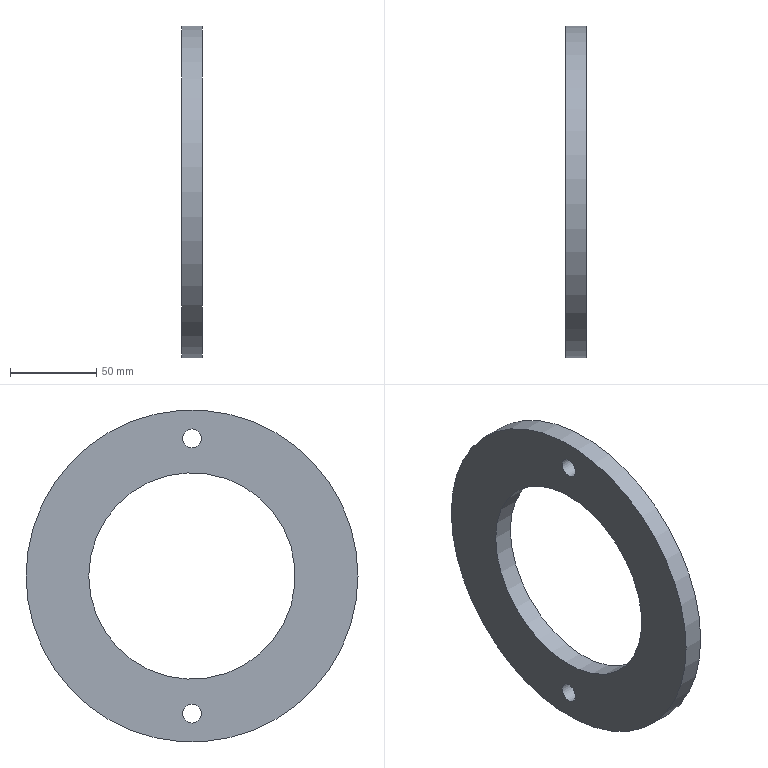Component | NX | LOCKING_PLATE | 1 solid | 6 faces | box 12 x 193 x 193 mm | volume 213066 mm3 | cylinder 4 | plane 2 | commonest cylinder face diameters 11 x2 193 x1 120 x1
STEP:
#1=CARTESIAN_POINT('',(0.,0.,0.));
#2=DIRECTION('',(0.,0.,1.));
#3=DIRECTION('',(1.,0.,0.));
#4=AXIS2_PLACEMENT_3D('',#1,#2,#3);
#5=CARTESIAN_POINT('',(-75.,96.5,-0.));
#6=VERTEX_POINT('',#5);
#7=CARTESIAN_POINT('',(-75.,0.,-0.));
#8=DIRECTION('',(1.,0.,0.));
#9=DIRECTION('',(0.,1.,-0.));
#10=AXIS2_PLACEMENT_3D('',#7,#8,#9);
#11=CIRCLE('',#10,96.5);
#12=CARTESIAN_POINT('',(-75.,0.,-0.));
#13=DIRECTION('',(-1.,0.,0.));
#14=DIRECTION('',(0.,0.,1.));
#15=AXIS2_PLACEMENT_3D('',#12,#13,#14);
#16=CYLINDRICAL_SURFACE('',#15,96.5);
#17=CARTESIAN_POINT('',(7.854,0.));
#18=DIRECTION('',(-1.,0.));
#19=VECTOR('',#18,1.);
#20=LINE('',#17,#19);
#21=(GEOMETRIC_REPRESENTATION_CONTEXT(2)PARAMETRIC_REPRESENTATION_CONTEXT()REPRESENTATION_CONTEXT('',''));
#22=DEFINITIONAL_REPRESENTATION('',(#20),#21);
#23=PCURVE('',#16,#22);
#24=CARTESIAN_POINT('',(-75.,0.,-0.));
#25=DIRECTION('',(1.,0.,0.));
#26=DIRECTION('',(0.,0.,-1.));
#27=AXIS2_PLACEMENT_3D('',#24,#25,#26);
#28=PLANE('',#27);
#29=CARTESIAN_POINT('',(0.,0.));
#30=DIRECTION('',(0.,1.));
#31=AXIS2_PLACEMENT_2D('',#29,#30);
#32=CIRCLE('',#31,96.5);
#33=(GEOMETRIC_REPRESENTATION_CONTEXT(2)PARAMETRIC_REPRESENTATION_CONTEXT()REPRESENTATION_CONTEXT('',''));
#34=DEFINITIONAL_REPRESENTATION('',(#32),#33);
#35=PCURVE('',#28,#34);
#36=SURFACE_CURVE('',#11,(#23,#35),.PCURVE_S1.);
#37=EDGE_CURVE('',#6,#6,#36,.T.);
#38=ORIENTED_EDGE('',*,*,#37,.F.);
#39=CARTESIAN_POINT('',(-87.,96.5,-0.));
#40=VERTEX_POINT('',#39);
#41=CARTESIAN_POINT('',(-75.,96.5,-0.));
#42=CARTESIAN_POINT('',(-87.,96.5,-0.));
#43=B_SPLINE_CURVE_WITH_KNOTS('',1,(#41,#42),.UNSPECIFIED.,.F.,.F.,(2,2),(0.,12.),.PIECEWISE_BEZIER_KNOTS.);
#44=CARTESIAN_POINT('',(7.854,0.));
#45=DIRECTION('',(0.,1.));
#46=VECTOR('',#45,1.);
#47=LINE('',#44,#46);
#48=(GEOMETRIC_REPRESENTATION_CONTEXT(2)PARAMETRIC_REPRESENTATION_CONTEXT()REPRESENTATION_CONTEXT('',''));
#49=DEFINITIONAL_REPRESENTATION('',(#47),#48);
#50=PCURVE('',#16,#49);
#51=CARTESIAN_POINT('',(1.571,0.));
#52=DIRECTION('',(0.,1.));
#53=VECTOR('',#52,1.);
#54=LINE('',#51,#53);
#55=(GEOMETRIC_REPRESENTATION_CONTEXT(2)PARAMETRIC_REPRESENTATION_CONTEXT()REPRESENTATION_CONTEXT('',''));
#56=DEFINITIONAL_REPRESENTATION('',(#54),#55);
#57=PCURVE('',#16,#56);
#58=SEAM_CURVE('',#43,(#50,#57),.PCURVE_S1.);
#59=EDGE_CURVE('',#6,#40,#58,.T.);
#60=ORIENTED_EDGE('',*,*,#59,.T.);
#61=CARTESIAN_POINT('',(-87.,0.,-0.));
#62=DIRECTION('',(1.,0.,0.));
#63=DIRECTION('',(0.,1.,-0.));
#64=AXIS2_PLACEMENT_3D('',#61,#62,#63);
#65=CIRCLE('',#64,96.5);
#66=CARTESIAN_POINT('',(7.854,12.));
#67=DIRECTION('',(-1.,0.));
#68=VECTOR('',#67,1.);
#69=LINE('',#66,#68);
#70=(GEOMETRIC_REPRESENTATION_CONTEXT(2)PARAMETRIC_REPRESENTATION_CONTEXT()REPRESENTATION_CONTEXT('',''));
#71=DEFINITIONAL_REPRESENTATION('',(#69),#70);
#72=PCURVE('',#16,#71);
#73=CARTESIAN_POINT('',(-87.,0.,-0.));
#74=DIRECTION('',(1.,0.,0.));
#75=DIRECTION('',(0.,0.,-1.));
#76=AXIS2_PLACEMENT_3D('',#73,#74,#75);
#77=PLANE('',#76);
#78=CARTESIAN_POINT('',(0.,0.));
#79=DIRECTION('',(0.,1.));
#80=AXIS2_PLACEMENT_2D('',#78,#79);
#81=CIRCLE('',#80,96.5);
#82=(GEOMETRIC_REPRESENTATION_CONTEXT(2)PARAMETRIC_REPRESENTATION_CONTEXT()REPRESENTATION_CONTEXT('',''));
#83=DEFINITIONAL_REPRESENTATION('',(#81),#82);
#84=PCURVE('',#77,#83);
#85=SURFACE_CURVE('',#65,(#72,#84),.PCURVE_S1.);
#86=EDGE_CURVE('',#40,#40,#85,.T.);
#87=ORIENTED_EDGE('',*,*,#86,.T.);
#88=ORIENTED_EDGE('',*,*,#59,.F.);
#89=EDGE_LOOP('',(#38,#60,#87,#88));
#90=FACE_BOUND('',#89,.T.);
#91=ADVANCED_FACE('',(#90),#16,.T.);
#92=CARTESIAN_POINT('',(-75.,60.,-0.));
#93=VERTEX_POINT('',#92);
#94=CARTESIAN_POINT('',(-75.,0.,-0.));
#95=DIRECTION('',(1.,0.,0.));
#96=DIRECTION('',(0.,1.,-0.));
#97=AXIS2_PLACEMENT_3D('',#94,#95,#96);
#98=CIRCLE('',#97,60.);
#99=CARTESIAN_POINT('',(-75.,0.,-0.));
#100=DIRECTION('',(-1.,0.,0.));
#101=DIRECTION('',(0.,0.,1.));
#102=AXIS2_PLACEMENT_3D('',#99,#100,#101);
#103=CYLINDRICAL_SURFACE('',#102,60.);
#104=CARTESIAN_POINT('',(7.854,0.));
#105=DIRECTION('',(-1.,0.));
#106=VECTOR('',#105,1.);
#107=LINE('',#104,#106);
#108=(GEOMETRIC_REPRESENTATION_CONTEXT(2)PARAMETRIC_REPRESENTATION_CONTEXT()REPRESENTATION_CONTEXT('',''));
#109=DEFINITIONAL_REPRESENTATION('',(#107),#108);
#110=PCURVE('',#103,#109);
#111=CARTESIAN_POINT('',(0.,0.));
#112=DIRECTION('',(0.,1.));
#113=AXIS2_PLACEMENT_2D('',#111,#112);
#114=CIRCLE('',#113,60.);
#115=(GEOMETRIC_REPRESENTATION_CONTEXT(2)PARAMETRIC_REPRESENTATION_CONTEXT()REPRESENTATION_CONTEXT('',''));
#116=DEFINITIONAL_REPRESENTATION('',(#114),#115);
#117=PCURVE('',#28,#116);
#118=SURFACE_CURVE('',#98,(#110,#117),.PCURVE_S1.);
#119=EDGE_CURVE('',#93,#93,#118,.T.);
#120=ORIENTED_EDGE('',*,*,#119,.F.);
#121=CARTESIAN_POINT('',(-87.,60.,-0.));
#122=VERTEX_POINT('',#121);
#123=CARTESIAN_POINT('',(-75.,60.,-0.));
#124=CARTESIAN_POINT('',(-87.,60.,-0.));
#125=B_SPLINE_CURVE_WITH_KNOTS('',1,(#123,#124),.UNSPECIFIED.,.F.,.F.,(2,2),(0.,12.),.PIECEWISE_BEZIER_KNOTS.);
#126=CARTESIAN_POINT('',(7.854,0.));
#127=DIRECTION('',(0.,1.));
#128=VECTOR('',#127,1.);
#129=LINE('',#126,#128);
#130=(GEOMETRIC_REPRESENTATION_CONTEXT(2)PARAMETRIC_REPRESENTATION_CONTEXT()REPRESENTATION_CONTEXT('',''));
#131=DEFINITIONAL_REPRESENTATION('',(#129),#130);
#132=PCURVE('',#103,#131);
#133=CARTESIAN_POINT('',(1.571,0.));
#134=DIRECTION('',(0.,1.));
#135=VECTOR('',#134,1.);
#136=LINE('',#133,#135);
#137=(GEOMETRIC_REPRESENTATION_CONTEXT(2)PARAMETRIC_REPRESENTATION_CONTEXT()REPRESENTATION_CONTEXT('',''));
#138=DEFINITIONAL_REPRESENTATION('',(#136),#137);
#139=PCURVE('',#103,#138);
#140=SEAM_CURVE('',#125,(#132,#139),.PCURVE_S1.);
#141=EDGE_CURVE('',#93,#122,#140,.T.);
#142=ORIENTED_EDGE('',*,*,#141,.T.);
#143=CARTESIAN_POINT('',(-87.,0.,-0.));
#144=DIRECTION('',(1.,0.,0.));
#145=DIRECTION('',(0.,1.,-0.));
#146=AXIS2_PLACEMENT_3D('',#143,#144,#145);
#147=CIRCLE('',#146,60.);
#148=CARTESIAN_POINT('',(7.854,12.));
#149=DIRECTION('',(-1.,0.));
#150=VECTOR('',#149,1.);
#151=LINE('',#148,#150);
#152=(GEOMETRIC_REPRESENTATION_CONTEXT(2)PARAMETRIC_REPRESENTATION_CONTEXT()REPRESENTATION_CONTEXT('',''));
#153=DEFINITIONAL_REPRESENTATION('',(#151),#152);
#154=PCURVE('',#103,#153);
#155=CARTESIAN_POINT('',(0.,0.));
#156=DIRECTION('',(0.,1.));
#157=AXIS2_PLACEMENT_2D('',#155,#156);
#158=CIRCLE('',#157,60.);
#159=(GEOMETRIC_REPRESENTATION_CONTEXT(2)PARAMETRIC_REPRESENTATION_CONTEXT()REPRESENTATION_CONTEXT('',''));
#160=DEFINITIONAL_REPRESENTATION('',(#158),#159);
#161=PCURVE('',#77,#160);
#162=SURFACE_CURVE('',#147,(#154,#161),.PCURVE_S1.);
#163=EDGE_CURVE('',#122,#122,#162,.T.);
#164=ORIENTED_EDGE('',*,*,#163,.T.);
#165=ORIENTED_EDGE('',*,*,#141,.F.);
#166=EDGE_LOOP('',(#120,#142,#164,#165));
#167=FACE_BOUND('',#166,.F.);
#168=ADVANCED_FACE('',(#167),#103,.F.);
#169=CARTESIAN_POINT('',(-75.,0.,85.5));
#170=VERTEX_POINT('',#169);
#171=CARTESIAN_POINT('',(-75.,0.,80.));
#172=DIRECTION('',(-1.,0.,0.));
#173=DIRECTION('',(0.,0.,1.));
#174=AXIS2_PLACEMENT_3D('',#171,#172,#173);
#175=CIRCLE('',#174,5.5);
#176=CARTESIAN_POINT('',(-85.5,0.));
#177=CARTESIAN_POINT('',(-85.5,9.526));
#178=CARTESIAN_POINT('',(-77.25,4.763));
#179=CARTESIAN_POINT('',(-69.,0.));
#180=CARTESIAN_POINT('',(-77.25,-4.763));
#181=CARTESIAN_POINT('',(-85.5,-9.526));
#182=CARTESIAN_POINT('',(-85.5,0.));
#183=(BOUNDED_CURVE()B_SPLINE_CURVE(2,(#176,#177,#178,#179,#180,#181,#182),.UNSPECIFIED.,.T.,.F.)B_SPLINE_CURVE_WITH_KNOTS((1,2,2,2,2,1),(-2.094,0.,2.094,4.189,6.283,8.378),.UNSPECIFIED.)CURVE()GEOMETRIC_REPRESENTATION_ITEM()RATIONAL_B_SPLINE_CURVE((1.,0.5,1.,0.5,1.,0.5,1.))REPRESENTATION_ITEM(''));
#184=(GEOMETRIC_REPRESENTATION_CONTEXT(2)PARAMETRIC_REPRESENTATION_CONTEXT()REPRESENTATION_CONTEXT('',''));
#185=DEFINITIONAL_REPRESENTATION('',(#183),#184);
#186=PCURVE('',#28,#185);
#187=CARTESIAN_POINT('',(-75.,0.,80.));
#188=DIRECTION('',(-1.,0.,0.));
#189=DIRECTION('',(0.,0.,1.));
#190=AXIS2_PLACEMENT_3D('',#187,#188,#189);
#191=CYLINDRICAL_SURFACE('',#190,5.5);
#192=CARTESIAN_POINT('',(0.,0.));
#193=DIRECTION('',(1.,0.));
#194=VECTOR('',#193,1.);
#195=LINE('',#192,#194);
#196=(GEOMETRIC_REPRESENTATION_CONTEXT(2)PARAMETRIC_REPRESENTATION_CONTEXT()REPRESENTATION_CONTEXT('',''));
#197=DEFINITIONAL_REPRESENTATION('',(#195),#196);
#198=PCURVE('',#191,#197);
#199=SURFACE_CURVE('',#175,(#186,#198),.PCURVE_S1.);
#200=EDGE_CURVE('',#170,#170,#199,.T.);
#201=ORIENTED_EDGE('',*,*,#200,.T.);
#202=EDGE_LOOP('',(#201));
#203=FACE_BOUND('',#202,.T.);
#204=CARTESIAN_POINT('',(-75.,0.,-74.5));
#205=VERTEX_POINT('',#204);
#206=CARTESIAN_POINT('',(-75.,0.,-80.));
#207=DIRECTION('',(-1.,0.,0.));
#208=DIRECTION('',(0.,0.,1.));
#209=AXIS2_PLACEMENT_3D('',#206,#207,#208);
#210=CIRCLE('',#209,5.5);
#211=CARTESIAN_POINT('',(74.5,0.));
#212=CARTESIAN_POINT('',(74.5,9.526));
#213=CARTESIAN_POINT('',(82.75,4.763));
#214=CARTESIAN_POINT('',(91.,0.));
#215=CARTESIAN_POINT('',(82.75,-4.763));
#216=CARTESIAN_POINT('',(74.5,-9.526));
#217=CARTESIAN_POINT('',(74.5,0.));
#218=(BOUNDED_CURVE()B_SPLINE_CURVE(2,(#211,#212,#213,#214,#215,#216,#217),.UNSPECIFIED.,.T.,.F.)B_SPLINE_CURVE_WITH_KNOTS((1,2,2,2,2,1),(-2.094,0.,2.094,4.189,6.283,8.378),.UNSPECIFIED.)CURVE()GEOMETRIC_REPRESENTATION_ITEM()RATIONAL_B_SPLINE_CURVE((1.,0.5,1.,0.5,1.,0.5,1.))REPRESENTATION_ITEM(''));
#219=(GEOMETRIC_REPRESENTATION_CONTEXT(2)PARAMETRIC_REPRESENTATION_CONTEXT()REPRESENTATION_CONTEXT('',''));
#220=DEFINITIONAL_REPRESENTATION('',(#218),#219);
#221=PCURVE('',#28,#220);
#222=CARTESIAN_POINT('',(-75.,0.,-80.));
#223=DIRECTION('',(-1.,0.,0.));
#224=DIRECTION('',(0.,0.,1.));
#225=AXIS2_PLACEMENT_3D('',#222,#223,#224);
#226=CYLINDRICAL_SURFACE('',#225,5.5);
#227=CARTESIAN_POINT('',(0.,0.));
#228=DIRECTION('',(1.,0.));
#229=VECTOR('',#228,1.);
#230=LINE('',#227,#229);
#231=(GEOMETRIC_REPRESENTATION_CONTEXT(2)PARAMETRIC_REPRESENTATION_CONTEXT()REPRESENTATION_CONTEXT('',''));
#232=DEFINITIONAL_REPRESENTATION('',(#230),#231);
#233=PCURVE('',#226,#232);
#234=SURFACE_CURVE('',#210,(#221,#233),.PCURVE_S1.);
#235=EDGE_CURVE('',#205,#205,#234,.T.);
#236=ORIENTED_EDGE('',*,*,#235,.T.);
#237=EDGE_LOOP('',(#236));
#238=FACE_BOUND('',#237,.T.);
#239=ORIENTED_EDGE('',*,*,#37,.T.);
#240=EDGE_LOOP('',(#239));
#241=FACE_BOUND('',#240,.T.);
#242=ORIENTED_EDGE('',*,*,#119,.F.);
#243=EDGE_LOOP('',(#242));
#244=FACE_BOUND('',#243,.T.);
#245=ADVANCED_FACE('',(#203,#238,#241,#244),#28,.T.);
#246=CARTESIAN_POINT('',(-87.,0.,74.5));
#247=VERTEX_POINT('',#246);
#248=CARTESIAN_POINT('',(-87.,0.,85.5));
#249=VERTEX_POINT('',#248);
#250=CARTESIAN_POINT('',(-87.,0.,80.));
#251=DIRECTION('',(1.,0.,0.));
#252=DIRECTION('',(0.,0.,-1.));
#253=AXIS2_PLACEMENT_3D('',#250,#251,#252);
#254=CIRCLE('',#253,5.5);
#255=CARTESIAN_POINT('',(-80.,0.));
#256=DIRECTION('',(1.,0.));
#257=AXIS2_PLACEMENT_2D('',#255,#256);
#258=CIRCLE('',#257,5.5);
#259=(GEOMETRIC_REPRESENTATION_CONTEXT(2)PARAMETRIC_REPRESENTATION_CONTEXT()REPRESENTATION_CONTEXT('',''));
#260=DEFINITIONAL_REPRESENTATION('',(#258),#259);
#261=PCURVE('',#77,#260);
#262=CARTESIAN_POINT('',(3.142,12.));
#263=DIRECTION('',(-1.,0.));
#264=VECTOR('',#263,1.);
#265=LINE('',#262,#264);
#266=(GEOMETRIC_REPRESENTATION_CONTEXT(2)PARAMETRIC_REPRESENTATION_CONTEXT()REPRESENTATION_CONTEXT('',''));
#267=DEFINITIONAL_REPRESENTATION('',(#265),#266);
#268=PCURVE('',#191,#267);
#269=SURFACE_CURVE('',#254,(#261,#268),.PCURVE_S1.);
#270=EDGE_CURVE('',#247,#249,#269,.T.);
#271=ORIENTED_EDGE('',*,*,#270,.T.);
#272=CARTESIAN_POINT('',(-87.,0.,80.));
#273=DIRECTION('',(1.,0.,0.));
#274=DIRECTION('',(0.,0.,-1.));
#275=AXIS2_PLACEMENT_3D('',#272,#273,#274);
#276=CIRCLE('',#275,5.5);
#277=CARTESIAN_POINT('',(-80.,0.));
#278=DIRECTION('',(1.,0.));
#279=AXIS2_PLACEMENT_2D('',#277,#278);
#280=CIRCLE('',#279,5.5);
#281=(GEOMETRIC_REPRESENTATION_CONTEXT(2)PARAMETRIC_REPRESENTATION_CONTEXT()REPRESENTATION_CONTEXT('',''));
#282=DEFINITIONAL_REPRESENTATION('',(#280),#281);
#283=PCURVE('',#77,#282);
#284=CARTESIAN_POINT('',(9.425,12.));
#285=DIRECTION('',(-1.,0.));
#286=VECTOR('',#285,1.);
#287=LINE('',#284,#286);
#288=(GEOMETRIC_REPRESENTATION_CONTEXT(2)PARAMETRIC_REPRESENTATION_CONTEXT()REPRESENTATION_CONTEXT('',''));
#289=DEFINITIONAL_REPRESENTATION('',(#287),#288);
#290=PCURVE('',#191,#289);
#291=SURFACE_CURVE('',#276,(#283,#290),.PCURVE_S1.);
#292=EDGE_CURVE('',#249,#247,#291,.T.);
#293=ORIENTED_EDGE('',*,*,#292,.T.);
#294=EDGE_LOOP('',(#271,#293));
#295=FACE_BOUND('',#294,.T.);
#296=CARTESIAN_POINT('',(-87.,0.,-85.5));
#297=VERTEX_POINT('',#296);
#298=CARTESIAN_POINT('',(-87.,0.,-74.5));
#299=VERTEX_POINT('',#298);
#300=CARTESIAN_POINT('',(-87.,0.,-80.));
#301=DIRECTION('',(1.,0.,0.));
#302=DIRECTION('',(0.,0.,-1.));
#303=AXIS2_PLACEMENT_3D('',#300,#301,#302);
#304=CIRCLE('',#303,5.5);
#305=CARTESIAN_POINT('',(80.,0.));
#306=DIRECTION('',(1.,0.));
#307=AXIS2_PLACEMENT_2D('',#305,#306);
#308=CIRCLE('',#307,5.5);
#309=(GEOMETRIC_REPRESENTATION_CONTEXT(2)PARAMETRIC_REPRESENTATION_CONTEXT()REPRESENTATION_CONTEXT('',''));
#310=DEFINITIONAL_REPRESENTATION('',(#308),#309);
#311=PCURVE('',#77,#310);
#312=CARTESIAN_POINT('',(3.142,12.));
#313=DIRECTION('',(-1.,0.));
#314=VECTOR('',#313,1.);
#315=LINE('',#312,#314);
#316=(GEOMETRIC_REPRESENTATION_CONTEXT(2)PARAMETRIC_REPRESENTATION_CONTEXT()REPRESENTATION_CONTEXT('',''));
#317=DEFINITIONAL_REPRESENTATION('',(#315),#316);
#318=PCURVE('',#226,#317);
#319=SURFACE_CURVE('',#304,(#311,#318),.PCURVE_S1.);
#320=EDGE_CURVE('',#297,#299,#319,.T.);
#321=ORIENTED_EDGE('',*,*,#320,.T.);
#322=CARTESIAN_POINT('',(-87.,0.,-80.));
#323=DIRECTION('',(1.,0.,0.));
#324=DIRECTION('',(0.,0.,-1.));
#325=AXIS2_PLACEMENT_3D('',#322,#323,#324);
#326=CIRCLE('',#325,5.5);
#327=CARTESIAN_POINT('',(80.,0.));
#328=DIRECTION('',(1.,0.));
#329=AXIS2_PLACEMENT_2D('',#327,#328);
#330=CIRCLE('',#329,5.5);
#331=(GEOMETRIC_REPRESENTATION_CONTEXT(2)PARAMETRIC_REPRESENTATION_CONTEXT()REPRESENTATION_CONTEXT('',''));
#332=DEFINITIONAL_REPRESENTATION('',(#330),#331);
#333=PCURVE('',#77,#332);
#334=CARTESIAN_POINT('',(9.425,12.));
#335=DIRECTION('',(-1.,0.));
#336=VECTOR('',#335,1.);
#337=LINE('',#334,#336);
#338=(GEOMETRIC_REPRESENTATION_CONTEXT(2)PARAMETRIC_REPRESENTATION_CONTEXT()REPRESENTATION_CONTEXT('',''));
#339=DEFINITIONAL_REPRESENTATION('',(#337),#338);
#340=PCURVE('',#226,#339);
#341=SURFACE_CURVE('',#326,(#333,#340),.PCURVE_S1.);
#342=EDGE_CURVE('',#299,#297,#341,.T.);
#343=ORIENTED_EDGE('',*,*,#342,.T.);
#344=EDGE_LOOP('',(#321,#343));
#345=FACE_BOUND('',#344,.T.);
#346=ORIENTED_EDGE('',*,*,#86,.F.);
#347=EDGE_LOOP('',(#346));
#348=FACE_BOUND('',#347,.T.);
#349=ORIENTED_EDGE('',*,*,#163,.T.);
#350=EDGE_LOOP('',(#349));
#351=FACE_BOUND('',#350,.T.);
#352=ADVANCED_FACE('',(#295,#345,#348,#351),#77,.F.);
#353=ORIENTED_EDGE('',*,*,#235,.T.);
#354=CARTESIAN_POINT('',(-75.,0.,-74.5));
#355=CARTESIAN_POINT('',(-87.,0.,-74.5));
#356=B_SPLINE_CURVE_WITH_KNOTS('',1,(#354,#355),.UNSPECIFIED.,.F.,.F.,(2,2),(0.,12.),.PIECEWISE_BEZIER_KNOTS.);
#357=CARTESIAN_POINT('',(6.283,0.));
#358=DIRECTION('',(0.,1.));
#359=VECTOR('',#358,1.);
#360=LINE('',#357,#359);
#361=(GEOMETRIC_REPRESENTATION_CONTEXT(2)PARAMETRIC_REPRESENTATION_CONTEXT()REPRESENTATION_CONTEXT('',''));
#362=DEFINITIONAL_REPRESENTATION('',(#360),#361);
#363=PCURVE('',#226,#362);
#364=CARTESIAN_POINT('',(0.,0.));
#365=DIRECTION('',(0.,1.));
#366=VECTOR('',#365,1.);
#367=LINE('',#364,#366);
#368=(GEOMETRIC_REPRESENTATION_CONTEXT(2)PARAMETRIC_REPRESENTATION_CONTEXT()REPRESENTATION_CONTEXT('',''));
#369=DEFINITIONAL_REPRESENTATION('',(#367),#368);
#370=PCURVE('',#226,#369);
#371=SEAM_CURVE('',#356,(#363,#370),.PCURVE_S1.);
#372=EDGE_CURVE('',#205,#299,#371,.T.);
#373=ORIENTED_EDGE('',*,*,#372,.T.);
#374=ORIENTED_EDGE('',*,*,#342,.T.);
#375=ORIENTED_EDGE('',*,*,#320,.T.);
#376=ORIENTED_EDGE('',*,*,#372,.F.);
#377=EDGE_LOOP('',(#353,#373,#374,#375,#376));
#378=FACE_BOUND('',#377,.F.);
#379=ADVANCED_FACE('',(#378),#226,.F.);
#380=ORIENTED_EDGE('',*,*,#200,.T.);
#381=CARTESIAN_POINT('',(-75.,0.,85.5));
#382=CARTESIAN_POINT('',(-87.,0.,85.5));
#383=B_SPLINE_CURVE_WITH_KNOTS('',1,(#381,#382),.UNSPECIFIED.,.F.,.F.,(2,2),(0.,12.),.PIECEWISE_BEZIER_KNOTS.);
#384=CARTESIAN_POINT('',(6.283,0.));
#385=DIRECTION('',(0.,1.));
#386=VECTOR('',#385,1.);
#387=LINE('',#384,#386);
#388=(GEOMETRIC_REPRESENTATION_CONTEXT(2)PARAMETRIC_REPRESENTATION_CONTEXT()REPRESENTATION_CONTEXT('',''));
#389=DEFINITIONAL_REPRESENTATION('',(#387),#388);
#390=PCURVE('',#191,#389);
#391=CARTESIAN_POINT('',(0.,0.));
#392=DIRECTION('',(0.,1.));
#393=VECTOR('',#392,1.);
#394=LINE('',#391,#393);
#395=(GEOMETRIC_REPRESENTATION_CONTEXT(2)PARAMETRIC_REPRESENTATION_CONTEXT()REPRESENTATION_CONTEXT('',''));
#396=DEFINITIONAL_REPRESENTATION('',(#394),#395);
#397=PCURVE('',#191,#396);
#398=SEAM_CURVE('',#383,(#390,#397),.PCURVE_S1.);
#399=EDGE_CURVE('',#170,#249,#398,.T.);
#400=ORIENTED_EDGE('',*,*,#399,.T.);
#401=ORIENTED_EDGE('',*,*,#292,.T.);
#402=ORIENTED_EDGE('',*,*,#270,.T.);
#403=ORIENTED_EDGE('',*,*,#399,.F.);
#404=EDGE_LOOP('',(#380,#400,#401,#402,#403));
#405=FACE_BOUND('',#404,.F.);
#406=ADVANCED_FACE('',(#405),#191,.F.);
#407=CLOSED_SHELL('',(#91,#168,#245,#352,#379,#406));
#408=MANIFOLD_SOLID_BREP('',#407);
#409=(LENGTH_UNIT()NAMED_UNIT(*)SI_UNIT(.MILLI.,.METRE.));
#410=UNCERTAINTY_MEASURE_WITH_UNIT(LENGTH_MEASURE(0.000005),#409,'','');
#411=(NAMED_UNIT(*)PLANE_ANGLE_UNIT()SI_UNIT($,.RADIAN.));
#412=(NAMED_UNIT(*)SI_UNIT($,.STERADIAN.)SOLID_ANGLE_UNIT());
#413=(GEOMETRIC_REPRESENTATION_CONTEXT(3)GLOBAL_UNCERTAINTY_ASSIGNED_CONTEXT((#410))GLOBAL_UNIT_ASSIGNED_CONTEXT((#409,#411,#412))REPRESENTATION_CONTEXT('',''));
#414=ADVANCED_BREP_SHAPE_REPRESENTATION('',(#4,#408),#413);